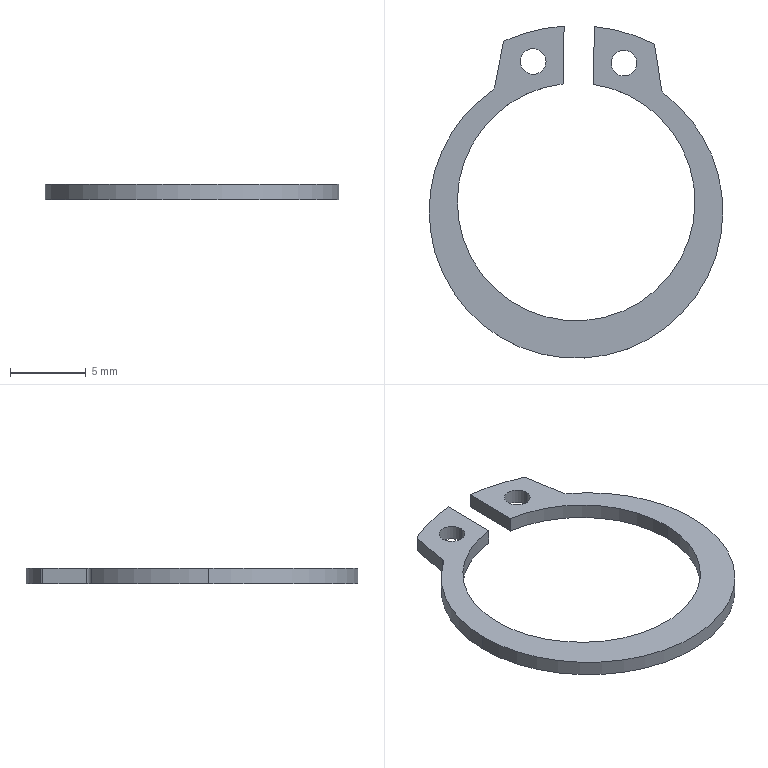Component | SolidWorks | HopperAssembly-1_20211103-210426-70669.STEP-1_-_-_-1.STEP-1_GB894_1-86_A_17.STEP-1 | 1 solid | 22 faces | box 19.4 x 21.94 x 1 mm | volume 118 mm3 | cylinder 16 | plane 6 | commonest cylinder face diameters 1.7 x4 19.4 x3 15.7 x3 1 x2 0.4 x2 23.3 x2
STEP:
#1=COLOUR_RGB('',0.7922,0.8196,0.9333);
#2=FILL_AREA_STYLE_COLOUR('',#1);
#3=FILL_AREA_STYLE('',(#2));
#4=SURFACE_STYLE_FILL_AREA(#3);
#5=SURFACE_SIDE_STYLE('',(#4));
#6=SURFACE_STYLE_USAGE(.BOTH.,#5);
#7=PRESENTATION_STYLE_ASSIGNMENT((#6));
#8=CARTESIAN_POINT('',(-104.551,33.416,-15.649));
#9=VERTEX_POINT('',#8);
#10=CARTESIAN_POINT('',(-104.484,33.414,-15.649));
#11=VERTEX_POINT('',#10);
#12=CARTESIAN_POINT('',(-104.517,33.415,-15.649));
#13=DIRECTION('',(0.,0.,-1.));
#14=DIRECTION('',(0.9998,-0.01747,0.));
#15=AXIS2_PLACEMENT_3D('',#12,#13,#14);
#16=CIRCLE('',#15,0.03346);
#17=EDGE_CURVE('',#9,#11,#16,.T.);
#18=ORIENTED_EDGE('',*,*,#17,.T.);
#19=CARTESIAN_POINT('',(-104.517,33.415,-15.649));
#20=DIRECTION('',(0.,0.,-1.));
#21=DIRECTION('',(0.9998,-0.01747,0.));
#22=AXIS2_PLACEMENT_3D('',#19,#20,#21);
#23=CIRCLE('',#22,0.03346);
#24=EDGE_CURVE('',#11,#9,#23,.T.);
#25=ORIENTED_EDGE('',*,*,#24,.T.);
#26=EDGE_LOOP('',(#18,#25));
#27=FACE_BOUND('',#26,.T.);
#28=CARTESIAN_POINT('',(-104.315,33.411,-15.649));
#29=VERTEX_POINT('',#28);
#30=CARTESIAN_POINT('',(-104.248,33.41,-15.649));
#31=VERTEX_POINT('',#30);
#32=CARTESIAN_POINT('',(-104.281,33.411,-15.649));
#33=DIRECTION('',(0.,0.,-1.));
#34=DIRECTION('',(-0.9998,0.01747,0.));
#35=AXIS2_PLACEMENT_3D('',#32,#33,#34);
#36=CIRCLE('',#35,0.03346);
#37=EDGE_CURVE('',#29,#31,#36,.T.);
#38=ORIENTED_EDGE('',*,*,#37,.T.);
#39=CARTESIAN_POINT('',(-104.281,33.411,-15.649));
#40=DIRECTION('',(0.,0.,-1.));
#41=DIRECTION('',(-0.9998,0.01747,0.));
#42=AXIS2_PLACEMENT_3D('',#39,#40,#41);
#43=CIRCLE('',#42,0.03346);
#44=EDGE_CURVE('',#31,#29,#43,.T.);
#45=ORIENTED_EDGE('',*,*,#44,.T.);
#46=EDGE_LOOP('',(#38,#45));
#47=FACE_BOUND('',#46,.T.);
#48=CARTESIAN_POINT('',(-104.625,33.338,-15.649));
#49=VERTEX_POINT('',#48);
#50=CARTESIAN_POINT('',(-104.617,33.35,-15.649));
#51=VERTEX_POINT('',#50);
#52=CARTESIAN_POINT('',(-104.637,33.354,-15.649));
#53=DIRECTION('',(-0.,-0.,1.));
#54=DIRECTION('',(0.9998,-0.01747,0.));
#55=AXIS2_PLACEMENT_3D('',#52,#53,#54);
#56=CIRCLE('',#55,0.01969);
#57=EDGE_CURVE('',#49,#51,#56,.T.);
#58=ORIENTED_EDGE('',*,*,#57,.F.);
#59=CARTESIAN_POINT('',(-104.788,33.032,-15.649));
#60=VERTEX_POINT('',#59);
#61=CARTESIAN_POINT('',(-104.406,33.025,-15.649));
#62=DIRECTION('',(0.,0.,-1.));
#63=DIRECTION('',(0.9998,-0.01747,0.));
#64=AXIS2_PLACEMENT_3D('',#61,#62,#63);
#65=CIRCLE('',#64,0.3819);
#66=EDGE_CURVE('',#60,#49,#65,.T.);
#67=ORIENTED_EDGE('',*,*,#66,.F.);
#68=CARTESIAN_POINT('',(-104.024,33.019,-15.649));
#69=VERTEX_POINT('',#68);
#70=CARTESIAN_POINT('',(-104.406,33.025,-15.649));
#71=DIRECTION('',(0.,0.,-1.));
#72=DIRECTION('',(0.9998,-0.01747,0.));
#73=AXIS2_PLACEMENT_3D('',#70,#71,#72);
#74=CIRCLE('',#73,0.3819);
#75=EDGE_CURVE('',#69,#60,#74,.T.);
#76=ORIENTED_EDGE('',*,*,#75,.F.);
#77=CARTESIAN_POINT('',(-104.176,33.33,-15.649));
#78=VERTEX_POINT('',#77);
#79=CARTESIAN_POINT('',(-104.406,33.025,-15.649));
#80=DIRECTION('',(0.,0.,-1.));
#81=DIRECTION('',(0.9998,-0.01747,0.));
#82=AXIS2_PLACEMENT_3D('',#79,#80,#81);
#83=CIRCLE('',#82,0.3819);
#84=EDGE_CURVE('',#78,#69,#83,.T.);
#85=ORIENTED_EDGE('',*,*,#84,.F.);
#86=CARTESIAN_POINT('',(-104.184,33.343,-15.649));
#87=VERTEX_POINT('',#86);
#88=CARTESIAN_POINT('',(-104.164,33.346,-15.649));
#89=DIRECTION('',(-0.,-0.,1.));
#90=DIRECTION('',(-0.9998,0.01747,0.));
#91=AXIS2_PLACEMENT_3D('',#88,#89,#90);
#92=CIRCLE('',#91,0.01969);
#93=EDGE_CURVE('',#87,#78,#92,.T.);
#94=ORIENTED_EDGE('',*,*,#93,.F.);
#95=CARTESIAN_POINT('',(-104.202,33.457,-15.649));
#96=VERTEX_POINT('',#95);
#97=CARTESIAN_POINT('',(-104.184,33.343,-15.649));
#98=DIRECTION('',(0.1564,-0.9877,-0.));
#99=VECTOR('',#98,39.37);
#100=LINE('',#97,#99);
#101=EDGE_CURVE('',#96,#87,#100,.T.);
#102=ORIENTED_EDGE('',*,*,#101,.F.);
#103=CARTESIAN_POINT('',(-104.206,33.463,-15.649));
#104=VERTEX_POINT('',#103);
#105=CARTESIAN_POINT('',(-104.209,33.456,-15.649));
#106=DIRECTION('',(0.,0.,-1.));
#107=DIRECTION('',(0.9998,-0.01747,0.));
#108=AXIS2_PLACEMENT_3D('',#105,#106,#107);
#109=CIRCLE('',#108,0.007874);
#110=EDGE_CURVE('',#104,#96,#109,.T.);
#111=ORIENTED_EDGE('',*,*,#110,.F.);
#112=CARTESIAN_POINT('',(-104.358,33.506,-15.649));
#113=VERTEX_POINT('',#112);
#114=CARTESIAN_POINT('',(-104.406,33.05,-15.649));
#115=DIRECTION('',(0.,0.,-1.));
#116=DIRECTION('',(0.9998,-0.01747,0.));
#117=AXIS2_PLACEMENT_3D('',#114,#115,#116);
#118=CIRCLE('',#117,0.4587);
#119=EDGE_CURVE('',#113,#104,#118,.T.);
#120=ORIENTED_EDGE('',*,*,#119,.F.);
#121=CARTESIAN_POINT('',(-104.361,33.356,-15.649));
#122=VERTEX_POINT('',#121);
#123=CARTESIAN_POINT('',(-104.361,33.356,-15.649));
#124=DIRECTION('',(0.01747,0.9998,0.));
#125=VECTOR('',#124,39.37);
#126=LINE('',#123,#125);
#127=EDGE_CURVE('',#122,#113,#126,.T.);
#128=ORIENTED_EDGE('',*,*,#127,.F.);
#129=CARTESIAN_POINT('',(-104.097,33.044,-15.649));
#130=VERTEX_POINT('',#129);
#131=CARTESIAN_POINT('',(-104.406,33.05,-15.649));
#132=DIRECTION('',(-0.,-0.,1.));
#133=DIRECTION('',(0.9998,-0.01747,0.));
#134=AXIS2_PLACEMENT_3D('',#131,#132,#133);
#135=CIRCLE('',#134,0.3091);
#136=EDGE_CURVE('',#130,#122,#135,.T.);
#137=ORIENTED_EDGE('',*,*,#136,.F.);
#138=CARTESIAN_POINT('',(-104.715,33.055,-15.649));
#139=VERTEX_POINT('',#138);
#140=CARTESIAN_POINT('',(-104.406,33.05,-15.649));
#141=DIRECTION('',(-0.,-0.,1.));
#142=DIRECTION('',(0.9998,-0.01747,0.));
#143=AXIS2_PLACEMENT_3D('',#140,#141,#142);
#144=CIRCLE('',#143,0.3091);
#145=EDGE_CURVE('',#139,#130,#144,.T.);
#146=ORIENTED_EDGE('',*,*,#145,.F.);
#147=CARTESIAN_POINT('',(-104.44,33.357,-15.649));
#148=VERTEX_POINT('',#147);
#149=CARTESIAN_POINT('',(-104.406,33.05,-15.649));
#150=DIRECTION('',(-0.,-0.,1.));
#151=DIRECTION('',(0.9998,-0.01747,0.));
#152=AXIS2_PLACEMENT_3D('',#149,#150,#151);
#153=CIRCLE('',#152,0.3091);
#154=EDGE_CURVE('',#148,#139,#153,.T.);
#155=ORIENTED_EDGE('',*,*,#154,.F.);
#156=CARTESIAN_POINT('',(-104.437,33.507,-15.649));
#157=VERTEX_POINT('',#156);
#158=CARTESIAN_POINT('',(-104.44,33.357,-15.649));
#159=DIRECTION('',(-0.01747,-0.9998,-0.));
#160=VECTOR('',#159,39.37);
#161=LINE('',#158,#160);
#162=EDGE_CURVE('',#157,#148,#161,.T.);
#163=ORIENTED_EDGE('',*,*,#162,.F.);
#164=CARTESIAN_POINT('',(-104.591,33.469,-15.649));
#165=VERTEX_POINT('',#164);
#166=CARTESIAN_POINT('',(-104.406,33.05,-15.649));
#167=DIRECTION('',(0.,0.,-1.));
#168=DIRECTION('',(-0.9998,0.01747,0.));
#169=AXIS2_PLACEMENT_3D('',#166,#167,#168);
#170=CIRCLE('',#169,0.4587);
#171=EDGE_CURVE('',#165,#157,#170,.T.);
#172=ORIENTED_EDGE('',*,*,#171,.F.);
#173=CARTESIAN_POINT('',(-104.595,33.464,-15.649));
#174=VERTEX_POINT('',#173);
#175=CARTESIAN_POINT('',(-104.588,33.462,-15.649));
#176=DIRECTION('',(0.,0.,-1.));
#177=DIRECTION('',(-0.9998,0.01747,0.));
#178=AXIS2_PLACEMENT_3D('',#175,#176,#177);
#179=CIRCLE('',#178,0.007874);
#180=EDGE_CURVE('',#174,#165,#179,.T.);
#181=ORIENTED_EDGE('',*,*,#180,.F.);
#182=CARTESIAN_POINT('',(-104.617,33.35,-15.649));
#183=DIRECTION('',(0.1908,0.9816,0.));
#184=VECTOR('',#183,39.37);
#185=LINE('',#182,#184);
#186=EDGE_CURVE('',#51,#174,#185,.T.);
#187=ORIENTED_EDGE('',*,*,#186,.F.);
#188=EDGE_LOOP('',(#58,#67,#76,#85,#94,#102,#111,#120,#128,#137,#146,#155,#163,#172,#181,#187));
#189=FACE_OUTER_BOUND('',#188,.T.);
#190=CARTESIAN_POINT('',(-104.637,33.354,-15.649));
#191=DIRECTION('',(0.,0.,-1.));
#192=DIRECTION('',(0.9998,-0.01747,0.));
#193=AXIS2_PLACEMENT_3D('',#190,#191,#192);
#194=PLANE('',#193);
#195=ADVANCED_FACE('',(#27,#47,#189),#194,.F.);
#196=CARTESIAN_POINT('',(-104.248,33.41,-15.688));
#197=VERTEX_POINT('',#196);
#198=CARTESIAN_POINT('',(-104.248,33.41,-15.688));
#199=DIRECTION('',(-0.,-0.,1.));
#200=VECTOR('',#199,39.37);
#201=LINE('',#198,#200);
#202=EDGE_CURVE('',#197,#31,#201,.T.);
#203=ORIENTED_EDGE('',*,*,#202,.F.);
#204=CARTESIAN_POINT('',(-104.315,33.411,-15.688));
#205=VERTEX_POINT('',#204);
#206=CARTESIAN_POINT('',(-104.281,33.411,-15.688));
#207=DIRECTION('',(0.,0.,-1.));
#208=DIRECTION('',(-0.9998,0.01747,0.));
#209=AXIS2_PLACEMENT_3D('',#206,#207,#208);
#210=CIRCLE('',#209,0.03346);
#211=EDGE_CURVE('',#197,#205,#210,.T.);
#212=ORIENTED_EDGE('',*,*,#211,.T.);
#213=CARTESIAN_POINT('',(-104.315,33.411,-15.688));
#214=DIRECTION('',(-0.,-0.,1.));
#215=VECTOR('',#214,39.37);
#216=LINE('',#213,#215);
#217=EDGE_CURVE('',#205,#29,#216,.T.);
#218=ORIENTED_EDGE('',*,*,#217,.T.);
#219=ORIENTED_EDGE('',*,*,#44,.F.);
#220=EDGE_LOOP('',(#203,#212,#218,#219));
#221=FACE_OUTER_BOUND('',#220,.T.);
#222=CARTESIAN_POINT('',(-104.281,33.411,-15.688));
#223=DIRECTION('',(-0.,-0.,1.));
#224=DIRECTION('',(-0.9998,0.01747,0.));
#225=AXIS2_PLACEMENT_3D('',#222,#223,#224);
#226=CYLINDRICAL_SURFACE('',#225,0.03346);
#227=ADVANCED_FACE('',(#221),#226,.F.);
#228=CARTESIAN_POINT('',(-104.484,33.414,-15.688));
#229=VERTEX_POINT('',#228);
#230=CARTESIAN_POINT('',(-104.484,33.414,-15.688));
#231=DIRECTION('',(-0.,-0.,1.));
#232=VECTOR('',#231,39.37);
#233=LINE('',#230,#232);
#234=EDGE_CURVE('',#229,#11,#233,.T.);
#235=ORIENTED_EDGE('',*,*,#234,.F.);
#236=CARTESIAN_POINT('',(-104.551,33.416,-15.688));
#237=VERTEX_POINT('',#236);
#238=CARTESIAN_POINT('',(-104.517,33.415,-15.688));
#239=DIRECTION('',(0.,0.,-1.));
#240=DIRECTION('',(0.9998,-0.01747,0.));
#241=AXIS2_PLACEMENT_3D('',#238,#239,#240);
#242=CIRCLE('',#241,0.03346);
#243=EDGE_CURVE('',#229,#237,#242,.T.);
#244=ORIENTED_EDGE('',*,*,#243,.T.);
#245=CARTESIAN_POINT('',(-104.551,33.416,-15.688));
#246=DIRECTION('',(-0.,-0.,1.));
#247=VECTOR('',#246,39.37);
#248=LINE('',#245,#247);
#249=EDGE_CURVE('',#237,#9,#248,.T.);
#250=ORIENTED_EDGE('',*,*,#249,.T.);
#251=ORIENTED_EDGE('',*,*,#24,.F.);
#252=EDGE_LOOP('',(#235,#244,#250,#251));
#253=FACE_OUTER_BOUND('',#252,.T.);
#254=CARTESIAN_POINT('',(-104.517,33.415,-15.688));
#255=DIRECTION('',(-0.,-0.,1.));
#256=DIRECTION('',(-0.9998,0.01747,0.));
#257=AXIS2_PLACEMENT_3D('',#254,#255,#256);
#258=CYLINDRICAL_SURFACE('',#257,0.03346);
#259=ADVANCED_FACE('',(#253),#258,.F.);
#260=CARTESIAN_POINT('',(-104.024,33.019,-15.688));
#261=VERTEX_POINT('',#260);
#262=CARTESIAN_POINT('',(-104.024,33.019,-15.688));
#263=DIRECTION('',(-0.,-0.,1.));
#264=VECTOR('',#263,39.37);
#265=LINE('',#262,#264);
#266=EDGE_CURVE('',#261,#69,#265,.T.);
#267=ORIENTED_EDGE('',*,*,#266,.F.);
#268=CARTESIAN_POINT('',(-104.176,33.33,-15.688));
#269=VERTEX_POINT('',#268);
#270=CARTESIAN_POINT('',(-104.406,33.025,-15.688));
#271=DIRECTION('',(0.,0.,-1.));
#272=DIRECTION('',(0.9998,-0.01747,0.));
#273=AXIS2_PLACEMENT_3D('',#270,#271,#272);
#274=CIRCLE('',#273,0.3819);
#275=EDGE_CURVE('',#269,#261,#274,.T.);
#276=ORIENTED_EDGE('',*,*,#275,.F.);
#277=CARTESIAN_POINT('',(-104.176,33.33,-15.688));
#278=DIRECTION('',(-0.,-0.,1.));
#279=VECTOR('',#278,39.37);
#280=LINE('',#277,#279);
#281=EDGE_CURVE('',#269,#78,#280,.T.);
#282=ORIENTED_EDGE('',*,*,#281,.T.);
#283=ORIENTED_EDGE('',*,*,#84,.T.);
#284=EDGE_LOOP('',(#267,#276,#282,#283));
#285=FACE_OUTER_BOUND('',#284,.T.);
#286=CARTESIAN_POINT('',(-104.406,33.025,-15.688));
#287=DIRECTION('',(-0.,-0.,1.));
#288=DIRECTION('',(-0.9998,0.01747,0.));
#289=AXIS2_PLACEMENT_3D('',#286,#287,#288);
#290=CYLINDRICAL_SURFACE('',#289,0.3819);
#291=ADVANCED_FACE('',(#285),#290,.T.);
#292=CARTESIAN_POINT('',(-104.184,33.343,-15.688));
#293=VERTEX_POINT('',#292);
#294=CARTESIAN_POINT('',(-104.184,33.343,-15.688));
#295=DIRECTION('',(-0.,-0.,1.));
#296=VECTOR('',#295,39.37);
#297=LINE('',#294,#296);
#298=EDGE_CURVE('',#293,#87,#297,.T.);
#299=ORIENTED_EDGE('',*,*,#298,.T.);
#300=ORIENTED_EDGE('',*,*,#93,.T.);
#301=ORIENTED_EDGE('',*,*,#281,.F.);
#302=CARTESIAN_POINT('',(-104.164,33.346,-15.688));
#303=DIRECTION('',(-0.,-0.,1.));
#304=DIRECTION('',(-0.9998,0.01747,0.));
#305=AXIS2_PLACEMENT_3D('',#302,#303,#304);
#306=CIRCLE('',#305,0.01969);
#307=EDGE_CURVE('',#293,#269,#306,.T.);
#308=ORIENTED_EDGE('',*,*,#307,.F.);
#309=EDGE_LOOP('',(#299,#300,#301,#308));
#310=FACE_OUTER_BOUND('',#309,.T.);
#311=CARTESIAN_POINT('',(-104.164,33.346,-15.688));
#312=DIRECTION('',(-0.,-0.,1.));
#313=DIRECTION('',(-0.9998,0.01747,0.));
#314=AXIS2_PLACEMENT_3D('',#311,#312,#313);
#315=CYLINDRICAL_SURFACE('',#314,0.01969);
#316=ADVANCED_FACE('',(#310),#315,.F.);
#317=CARTESIAN_POINT('',(-104.202,33.457,-15.688));
#318=VERTEX_POINT('',#317);
#319=CARTESIAN_POINT('',(-104.202,33.457,-15.688));
#320=DIRECTION('',(-0.,-0.,1.));
#321=VECTOR('',#320,39.37);
#322=LINE('',#319,#321);
#323=EDGE_CURVE('',#318,#96,#322,.T.);
#324=ORIENTED_EDGE('',*,*,#323,.T.);
#325=ORIENTED_EDGE('',*,*,#101,.T.);
#326=ORIENTED_EDGE('',*,*,#298,.F.);
#327=CARTESIAN_POINT('',(-104.184,33.343,-15.688));
#328=DIRECTION('',(0.1564,-0.9877,-0.));
#329=VECTOR('',#328,39.37);
#330=LINE('',#327,#329);
#331=EDGE_CURVE('',#318,#293,#330,.T.);
#332=ORIENTED_EDGE('',*,*,#331,.F.);
#333=EDGE_LOOP('',(#324,#325,#326,#332));
#334=FACE_OUTER_BOUND('',#333,.T.);
#335=CARTESIAN_POINT('',(-104.184,33.343,-15.688));
#336=DIRECTION('',(-0.9877,-0.1564,-0.));
#337=DIRECTION('',(0.,0.,-1.));
#338=AXIS2_PLACEMENT_3D('',#335,#336,#337);
#339=PLANE('',#338);
#340=ADVANCED_FACE('',(#334),#339,.F.);
#341=CARTESIAN_POINT('',(-104.206,33.463,-15.688));
#342=VERTEX_POINT('',#341);
#343=CARTESIAN_POINT('',(-104.206,33.463,-15.688));
#344=DIRECTION('',(-0.,-0.,1.));
#345=VECTOR('',#344,39.37);
#346=LINE('',#343,#345);
#347=EDGE_CURVE('',#342,#104,#346,.T.);
#348=ORIENTED_EDGE('',*,*,#347,.T.);
#349=ORIENTED_EDGE('',*,*,#110,.T.);
#350=ORIENTED_EDGE('',*,*,#323,.F.);
#351=CARTESIAN_POINT('',(-104.209,33.456,-15.688));
#352=DIRECTION('',(0.,0.,-1.));
#353=DIRECTION('',(0.9998,-0.01747,0.));
#354=AXIS2_PLACEMENT_3D('',#351,#352,#353);
#355=CIRCLE('',#354,0.007874);
#356=EDGE_CURVE('',#342,#318,#355,.T.);
#357=ORIENTED_EDGE('',*,*,#356,.F.);
#358=EDGE_LOOP('',(#348,#349,#350,#357));
#359=FACE_OUTER_BOUND('',#358,.T.);
#360=CARTESIAN_POINT('',(-104.209,33.456,-15.688));
#361=DIRECTION('',(-0.,-0.,1.));
#362=DIRECTION('',(-0.9998,0.01747,0.));
#363=AXIS2_PLACEMENT_3D('',#360,#361,#362);
#364=CYLINDRICAL_SURFACE('',#363,0.007874);
#365=ADVANCED_FACE('',(#359),#364,.T.);
#366=CARTESIAN_POINT('',(-104.358,33.506,-15.688));
#367=VERTEX_POINT('',#366);
#368=CARTESIAN_POINT('',(-104.358,33.506,-15.688));
#369=DIRECTION('',(-0.,-0.,1.));
#370=VECTOR('',#369,39.37);
#371=LINE('',#368,#370);
#372=EDGE_CURVE('',#367,#113,#371,.T.);
#373=ORIENTED_EDGE('',*,*,#372,.T.);
#374=ORIENTED_EDGE('',*,*,#119,.T.);
#375=ORIENTED_EDGE('',*,*,#347,.F.);
#376=CARTESIAN_POINT('',(-104.406,33.05,-15.688));
#377=DIRECTION('',(0.,0.,-1.));
#378=DIRECTION('',(0.9998,-0.01747,0.));
#379=AXIS2_PLACEMENT_3D('',#376,#377,#378);
#380=CIRCLE('',#379,0.4587);
#381=EDGE_CURVE('',#367,#342,#380,.T.);
#382=ORIENTED_EDGE('',*,*,#381,.F.);
#383=EDGE_LOOP('',(#373,#374,#375,#382));
#384=FACE_OUTER_BOUND('',#383,.T.);
#385=CARTESIAN_POINT('',(-104.406,33.05,-15.688));
#386=DIRECTION('',(-0.,-0.,1.));
#387=DIRECTION('',(-0.9998,0.01747,0.));
#388=AXIS2_PLACEMENT_3D('',#385,#386,#387);
#389=CYLINDRICAL_SURFACE('',#388,0.4587);
#390=ADVANCED_FACE('',(#384),#389,.T.);
#391=CARTESIAN_POINT('',(-104.361,33.356,-15.688));
#392=VERTEX_POINT('',#391);
#393=CARTESIAN_POINT('',(-104.361,33.356,-15.688));
#394=DIRECTION('',(-0.,-0.,1.));
#395=VECTOR('',#394,39.37);
#396=LINE('',#393,#395);
#397=EDGE_CURVE('',#392,#122,#396,.T.);
#398=ORIENTED_EDGE('',*,*,#397,.T.);
#399=ORIENTED_EDGE('',*,*,#127,.T.);
#400=ORIENTED_EDGE('',*,*,#372,.F.);
#401=CARTESIAN_POINT('',(-104.361,33.356,-15.688));
#402=DIRECTION('',(0.01747,0.9998,0.));
#403=VECTOR('',#402,39.37);
#404=LINE('',#401,#403);
#405=EDGE_CURVE('',#392,#367,#404,.T.);
#406=ORIENTED_EDGE('',*,*,#405,.F.);
#407=EDGE_LOOP('',(#398,#399,#400,#406));
#408=FACE_OUTER_BOUND('',#407,.T.);
#409=CARTESIAN_POINT('',(-104.361,33.356,-15.688));
#410=DIRECTION('',(0.9998,-0.01747,0.));
#411=DIRECTION('',(-0.01747,-0.9998,-0.));
#412=AXIS2_PLACEMENT_3D('',#409,#410,#411);
#413=PLANE('',#412);
#414=ADVANCED_FACE('',(#408),#413,.F.);
#415=CARTESIAN_POINT('',(-104.715,33.055,-15.688));
#416=VERTEX_POINT('',#415);
#417=CARTESIAN_POINT('',(-104.715,33.055,-15.688));
#418=DIRECTION('',(-0.,-0.,1.));
#419=VECTOR('',#418,39.37);
#420=LINE('',#417,#419);
#421=EDGE_CURVE('',#416,#139,#420,.T.);
#422=ORIENTED_EDGE('',*,*,#421,.F.);
#423=CARTESIAN_POINT('',(-104.44,33.357,-15.688));
#424=VERTEX_POINT('',#423);
#425=CARTESIAN_POINT('',(-104.406,33.05,-15.688));
#426=DIRECTION('',(-0.,-0.,1.));
#427=DIRECTION('',(0.9998,-0.01747,0.));
#428=AXIS2_PLACEMENT_3D('',#425,#426,#427);
#429=CIRCLE('',#428,0.3091);
#430=EDGE_CURVE('',#424,#416,#429,.T.);
#431=ORIENTED_EDGE('',*,*,#430,.F.);
#432=CARTESIAN_POINT('',(-104.44,33.357,-15.688));
#433=DIRECTION('',(-0.,-0.,1.));
#434=VECTOR('',#433,39.37);
#435=LINE('',#432,#434);
#436=EDGE_CURVE('',#424,#148,#435,.T.);
#437=ORIENTED_EDGE('',*,*,#436,.T.);
#438=ORIENTED_EDGE('',*,*,#154,.T.);
#439=EDGE_LOOP('',(#422,#431,#437,#438));
#440=FACE_OUTER_BOUND('',#439,.T.);
#441=CARTESIAN_POINT('',(-104.406,33.05,-15.688));
#442=DIRECTION('',(-0.,-0.,1.));
#443=DIRECTION('',(-0.9998,0.01747,0.));
#444=AXIS2_PLACEMENT_3D('',#441,#442,#443);
#445=CYLINDRICAL_SURFACE('',#444,0.3091);
#446=ADVANCED_FACE('',(#440),#445,.F.);
#447=CARTESIAN_POINT('',(-104.437,33.507,-15.688));
#448=VERTEX_POINT('',#447);
#449=CARTESIAN_POINT('',(-104.437,33.507,-15.688));
#450=DIRECTION('',(-0.,-0.,1.));
#451=VECTOR('',#450,39.37);
#452=LINE('',#449,#451);
#453=EDGE_CURVE('',#448,#157,#452,.T.);
#454=ORIENTED_EDGE('',*,*,#453,.T.);
#455=ORIENTED_EDGE('',*,*,#162,.T.);
#456=ORIENTED_EDGE('',*,*,#436,.F.);
#457=CARTESIAN_POINT('',(-104.44,33.357,-15.688));
#458=DIRECTION('',(-0.01747,-0.9998,-0.));
#459=VECTOR('',#458,39.37);
#460=LINE('',#457,#459);
#461=EDGE_CURVE('',#448,#424,#460,.T.);
#462=ORIENTED_EDGE('',*,*,#461,.F.);
#463=EDGE_LOOP('',(#454,#455,#456,#462));
#464=FACE_OUTER_BOUND('',#463,.T.);
#465=CARTESIAN_POINT('',(-104.44,33.357,-15.688));
#466=DIRECTION('',(-0.9998,0.01747,-0.));
#467=DIRECTION('',(-0.01747,-0.9998,-0.));
#468=AXIS2_PLACEMENT_3D('',#465,#466,#467);
#469=PLANE('',#468);
#470=ADVANCED_FACE('',(#464),#469,.F.);
#471=CARTESIAN_POINT('',(-104.591,33.469,-15.688));
#472=VERTEX_POINT('',#471);
#473=CARTESIAN_POINT('',(-104.591,33.469,-15.688));
#474=DIRECTION('',(-0.,-0.,1.));
#475=VECTOR('',#474,39.37);
#476=LINE('',#473,#475);
#477=EDGE_CURVE('',#472,#165,#476,.T.);
#478=ORIENTED_EDGE('',*,*,#477,.T.);
#479=ORIENTED_EDGE('',*,*,#171,.T.);
#480=ORIENTED_EDGE('',*,*,#453,.F.);
#481=CARTESIAN_POINT('',(-104.406,33.05,-15.688));
#482=DIRECTION('',(0.,0.,-1.));
#483=DIRECTION('',(-0.9998,0.01747,0.));
#484=AXIS2_PLACEMENT_3D('',#481,#482,#483);
#485=CIRCLE('',#484,0.4587);
#486=EDGE_CURVE('',#472,#448,#485,.T.);
#487=ORIENTED_EDGE('',*,*,#486,.F.);
#488=EDGE_LOOP('',(#478,#479,#480,#487));
#489=FACE_OUTER_BOUND('',#488,.T.);
#490=CARTESIAN_POINT('',(-104.406,33.05,-15.688));
#491=DIRECTION('',(-0.,-0.,1.));
#492=DIRECTION('',(-0.9998,0.01747,0.));
#493=AXIS2_PLACEMENT_3D('',#490,#491,#492);
#494=CYLINDRICAL_SURFACE('',#493,0.4587);
#495=ADVANCED_FACE('',(#489),#494,.T.);
#496=CARTESIAN_POINT('',(-104.595,33.464,-15.688));
#497=VERTEX_POINT('',#496);
#498=CARTESIAN_POINT('',(-104.595,33.464,-15.688));
#499=DIRECTION('',(-0.,-0.,1.));
#500=VECTOR('',#499,39.37);
#501=LINE('',#498,#500);
#502=EDGE_CURVE('',#497,#174,#501,.T.);
#503=ORIENTED_EDGE('',*,*,#502,.T.);
#504=ORIENTED_EDGE('',*,*,#180,.T.);
#505=ORIENTED_EDGE('',*,*,#477,.F.);
#506=CARTESIAN_POINT('',(-104.588,33.462,-15.688));
#507=DIRECTION('',(0.,0.,-1.));
#508=DIRECTION('',(-0.9998,0.01747,0.));
#509=AXIS2_PLACEMENT_3D('',#506,#507,#508);
#510=CIRCLE('',#509,0.007874);
#511=EDGE_CURVE('',#497,#472,#510,.T.);
#512=ORIENTED_EDGE('',*,*,#511,.F.);
#513=EDGE_LOOP('',(#503,#504,#505,#512));
#514=FACE_OUTER_BOUND('',#513,.T.);
#515=CARTESIAN_POINT('',(-104.588,33.462,-15.688));
#516=DIRECTION('',(-0.,-0.,1.));
#517=DIRECTION('',(-0.9998,0.01747,0.));
#518=AXIS2_PLACEMENT_3D('',#515,#516,#517);
#519=CYLINDRICAL_SURFACE('',#518,0.007874);
#520=ADVANCED_FACE('',(#514),#519,.T.);
#521=CARTESIAN_POINT('',(-104.617,33.35,-15.688));
#522=VERTEX_POINT('',#521);
#523=CARTESIAN_POINT('',(-104.617,33.35,-15.688));
#524=DIRECTION('',(-0.,-0.,1.));
#525=VECTOR('',#524,39.37);
#526=LINE('',#523,#525);
#527=EDGE_CURVE('',#522,#51,#526,.T.);
#528=ORIENTED_EDGE('',*,*,#527,.T.);
#529=ORIENTED_EDGE('',*,*,#186,.T.);
#530=ORIENTED_EDGE('',*,*,#502,.F.);
#531=CARTESIAN_POINT('',(-104.617,33.35,-15.688));
#532=DIRECTION('',(0.1908,0.9816,0.));
#533=VECTOR('',#532,39.37);
#534=LINE('',#531,#533);
#535=EDGE_CURVE('',#522,#497,#534,.T.);
#536=ORIENTED_EDGE('',*,*,#535,.F.);
#537=EDGE_LOOP('',(#528,#529,#530,#536));
#538=FACE_OUTER_BOUND('',#537,.T.);
#539=CARTESIAN_POINT('',(-104.617,33.35,-15.688));
#540=DIRECTION('',(0.9816,-0.1908,0.));
#541=DIRECTION('',(-0.,-0.,1.));
#542=AXIS2_PLACEMENT_3D('',#539,#540,#541);
#543=PLANE('',#542);
#544=ADVANCED_FACE('',(#538),#543,.F.);
#545=CARTESIAN_POINT('',(-104.625,33.338,-15.688));
#546=VERTEX_POINT('',#545);
#547=CARTESIAN_POINT('',(-104.625,33.338,-15.688));
#548=DIRECTION('',(-0.,-0.,1.));
#549=VECTOR('',#548,39.37);
#550=LINE('',#547,#549);
#551=EDGE_CURVE('',#546,#49,#550,.T.);
#552=ORIENTED_EDGE('',*,*,#551,.T.);
#553=ORIENTED_EDGE('',*,*,#57,.T.);
#554=ORIENTED_EDGE('',*,*,#527,.F.);
#555=CARTESIAN_POINT('',(-104.637,33.354,-15.688));
#556=DIRECTION('',(-0.,-0.,1.));
#557=DIRECTION('',(0.9998,-0.01747,0.));
#558=AXIS2_PLACEMENT_3D('',#555,#556,#557);
#559=CIRCLE('',#558,0.01969);
#560=EDGE_CURVE('',#546,#522,#559,.T.);
#561=ORIENTED_EDGE('',*,*,#560,.F.);
#562=EDGE_LOOP('',(#552,#553,#554,#561));
#563=FACE_OUTER_BOUND('',#562,.T.);
#564=CARTESIAN_POINT('',(-104.637,33.354,-15.688));
#565=DIRECTION('',(-0.,-0.,1.));
#566=DIRECTION('',(-0.9998,0.01747,0.));
#567=AXIS2_PLACEMENT_3D('',#564,#565,#566);
#568=CYLINDRICAL_SURFACE('',#567,0.01969);
#569=ADVANCED_FACE('',(#563),#568,.F.);
#570=CARTESIAN_POINT('',(-104.281,33.411,-15.688));
#571=DIRECTION('',(0.,0.,-1.));
#572=DIRECTION('',(-0.9998,0.01747,0.));
#573=AXIS2_PLACEMENT_3D('',#570,#571,#572);
#574=CIRCLE('',#573,0.03346);
#575=EDGE_CURVE('',#205,#197,#574,.T.);
#576=ORIENTED_EDGE('',*,*,#575,.F.);
#577=ORIENTED_EDGE('',*,*,#211,.F.);
#578=EDGE_LOOP('',(#576,#577));
#579=FACE_BOUND('',#578,.T.);
#580=CARTESIAN_POINT('',(-104.517,33.415,-15.688));
#581=DIRECTION('',(0.,0.,-1.));
#582=DIRECTION('',(0.9998,-0.01747,0.));
#583=AXIS2_PLACEMENT_3D('',#580,#581,#582);
#584=CIRCLE('',#583,0.03346);
#585=EDGE_CURVE('',#237,#229,#584,.T.);
#586=ORIENTED_EDGE('',*,*,#585,.F.);
#587=ORIENTED_EDGE('',*,*,#243,.F.);
#588=EDGE_LOOP('',(#586,#587));
#589=FACE_BOUND('',#588,.T.);
#590=ORIENTED_EDGE('',*,*,#560,.T.);
#591=ORIENTED_EDGE('',*,*,#535,.T.);
#592=ORIENTED_EDGE('',*,*,#511,.T.);
#593=ORIENTED_EDGE('',*,*,#486,.T.);
#594=ORIENTED_EDGE('',*,*,#461,.T.);
#595=ORIENTED_EDGE('',*,*,#430,.T.);
#596=CARTESIAN_POINT('',(-104.097,33.044,-15.688));
#597=VERTEX_POINT('',#596);
#598=CARTESIAN_POINT('',(-104.406,33.05,-15.688));
#599=DIRECTION('',(-0.,-0.,1.));
#600=DIRECTION('',(0.9998,-0.01747,0.));
#601=AXIS2_PLACEMENT_3D('',#598,#599,#600);
#602=CIRCLE('',#601,0.3091);
#603=EDGE_CURVE('',#416,#597,#602,.T.);
#604=ORIENTED_EDGE('',*,*,#603,.T.);
#605=CARTESIAN_POINT('',(-104.406,33.05,-15.688));
#606=DIRECTION('',(-0.,-0.,1.));
#607=DIRECTION('',(0.9998,-0.01747,0.));
#608=AXIS2_PLACEMENT_3D('',#605,#606,#607);
#609=CIRCLE('',#608,0.3091);
#610=EDGE_CURVE('',#597,#392,#609,.T.);
#611=ORIENTED_EDGE('',*,*,#610,.T.);
#612=ORIENTED_EDGE('',*,*,#405,.T.);
#613=ORIENTED_EDGE('',*,*,#381,.T.);
#614=ORIENTED_EDGE('',*,*,#356,.T.);
#615=ORIENTED_EDGE('',*,*,#331,.T.);
#616=ORIENTED_EDGE('',*,*,#307,.T.);
#617=ORIENTED_EDGE('',*,*,#275,.T.);
#618=CARTESIAN_POINT('',(-104.788,33.032,-15.688));
#619=VERTEX_POINT('',#618);
#620=CARTESIAN_POINT('',(-104.406,33.025,-15.688));
#621=DIRECTION('',(0.,0.,-1.));
#622=DIRECTION('',(0.9998,-0.01747,0.));
#623=AXIS2_PLACEMENT_3D('',#620,#621,#622);
#624=CIRCLE('',#623,0.3819);
#625=EDGE_CURVE('',#261,#619,#624,.T.);
#626=ORIENTED_EDGE('',*,*,#625,.T.);
#627=CARTESIAN_POINT('',(-104.406,33.025,-15.688));
#628=DIRECTION('',(0.,0.,-1.));
#629=DIRECTION('',(0.9998,-0.01747,0.));
#630=AXIS2_PLACEMENT_3D('',#627,#628,#629);
#631=CIRCLE('',#630,0.3819);
#632=EDGE_CURVE('',#619,#546,#631,.T.);
#633=ORIENTED_EDGE('',*,*,#632,.T.);
#634=EDGE_LOOP('',(#590,#591,#592,#593,#594,#595,#604,#611,#612,#613,#614,#615,#616,#617,#626,#633));
#635=FACE_OUTER_BOUND('',#634,.T.);
#636=CARTESIAN_POINT('',(-104.637,33.354,-15.688));
#637=DIRECTION('',(0.,0.,-1.));
#638=DIRECTION('',(0.9998,-0.01747,0.));
#639=AXIS2_PLACEMENT_3D('',#636,#637,#638);
#640=PLANE('',#639);
#641=ADVANCED_FACE('',(#579,#589,#635),#640,.T.);
#642=CARTESIAN_POINT('',(-104.097,33.044,-15.688));
#643=DIRECTION('',(-0.,-0.,1.));
#644=VECTOR('',#643,39.37);
#645=LINE('',#642,#644);
#646=EDGE_CURVE('',#597,#130,#645,.T.);
#647=ORIENTED_EDGE('',*,*,#646,.F.);
#648=ORIENTED_EDGE('',*,*,#603,.F.);
#649=ORIENTED_EDGE('',*,*,#421,.T.);
#650=ORIENTED_EDGE('',*,*,#145,.T.);
#651=EDGE_LOOP('',(#647,#648,#649,#650));
#652=FACE_OUTER_BOUND('',#651,.T.);
#653=CARTESIAN_POINT('',(-104.406,33.05,-15.688));
#654=DIRECTION('',(-0.,-0.,1.));
#655=DIRECTION('',(-0.9998,0.01747,0.));
#656=AXIS2_PLACEMENT_3D('',#653,#654,#655);
#657=CYLINDRICAL_SURFACE('',#656,0.3091);
#658=ADVANCED_FACE('',(#652),#657,.F.);
#659=ORIENTED_EDGE('',*,*,#610,.F.);
#660=ORIENTED_EDGE('',*,*,#646,.T.);
#661=ORIENTED_EDGE('',*,*,#136,.T.);
#662=ORIENTED_EDGE('',*,*,#397,.F.);
#663=EDGE_LOOP('',(#659,#660,#661,#662));
#664=FACE_OUTER_BOUND('',#663,.T.);
#665=CARTESIAN_POINT('',(-104.406,33.05,-15.688));
#666=DIRECTION('',(-0.,-0.,1.));
#667=DIRECTION('',(-0.9998,0.01747,0.));
#668=AXIS2_PLACEMENT_3D('',#665,#666,#667);
#669=CYLINDRICAL_SURFACE('',#668,0.3091);
#670=ADVANCED_FACE('',(#664),#669,.F.);
#671=ORIENTED_EDGE('',*,*,#632,.F.);
#672=CARTESIAN_POINT('',(-104.788,33.032,-15.688));
#673=DIRECTION('',(-0.,-0.,1.));
#674=VECTOR('',#673,39.37);
#675=LINE('',#672,#674);
#676=EDGE_CURVE('',#619,#60,#675,.T.);
#677=ORIENTED_EDGE('',*,*,#676,.T.);
#678=ORIENTED_EDGE('',*,*,#66,.T.);
#679=ORIENTED_EDGE('',*,*,#551,.F.);
#680=EDGE_LOOP('',(#671,#677,#678,#679));
#681=FACE_OUTER_BOUND('',#680,.T.);
#682=CARTESIAN_POINT('',(-104.406,33.025,-15.688));
#683=DIRECTION('',(-0.,-0.,1.));
#684=DIRECTION('',(-0.9998,0.01747,0.));
#685=AXIS2_PLACEMENT_3D('',#682,#683,#684);
#686=CYLINDRICAL_SURFACE('',#685,0.3819);
#687=ADVANCED_FACE('',(#681),#686,.T.);
#688=ORIENTED_EDGE('',*,*,#625,.F.);
#689=ORIENTED_EDGE('',*,*,#266,.T.);
#690=ORIENTED_EDGE('',*,*,#75,.T.);
#691=ORIENTED_EDGE('',*,*,#676,.F.);
#692=EDGE_LOOP('',(#688,#689,#690,#691));
#693=FACE_OUTER_BOUND('',#692,.T.);
#694=CARTESIAN_POINT('',(-104.406,33.025,-15.688));
#695=DIRECTION('',(-0.,-0.,1.));
#696=DIRECTION('',(-0.9998,0.01747,0.));
#697=AXIS2_PLACEMENT_3D('',#694,#695,#696);
#698=CYLINDRICAL_SURFACE('',#697,0.3819);
#699=ADVANCED_FACE('',(#693),#698,.T.);
#700=ORIENTED_EDGE('',*,*,#585,.T.);
#701=ORIENTED_EDGE('',*,*,#234,.T.);
#702=ORIENTED_EDGE('',*,*,#17,.F.);
#703=ORIENTED_EDGE('',*,*,#249,.F.);
#704=EDGE_LOOP('',(#700,#701,#702,#703));
#705=FACE_OUTER_BOUND('',#704,.T.);
#706=CARTESIAN_POINT('',(-104.517,33.415,-15.688));
#707=DIRECTION('',(-0.,-0.,1.));
#708=DIRECTION('',(-0.9998,0.01747,0.));
#709=AXIS2_PLACEMENT_3D('',#706,#707,#708);
#710=CYLINDRICAL_SURFACE('',#709,0.03346);
#711=ADVANCED_FACE('',(#705),#710,.F.);
#712=ORIENTED_EDGE('',*,*,#575,.T.);
#713=ORIENTED_EDGE('',*,*,#202,.T.);
#714=ORIENTED_EDGE('',*,*,#37,.F.);
#715=ORIENTED_EDGE('',*,*,#217,.F.);
#716=EDGE_LOOP('',(#712,#713,#714,#715));
#717=FACE_OUTER_BOUND('',#716,.T.);
#718=CARTESIAN_POINT('',(-104.281,33.411,-15.688));
#719=DIRECTION('',(-0.,-0.,1.));
#720=DIRECTION('',(-0.9998,0.01747,0.));
#721=AXIS2_PLACEMENT_3D('',#718,#719,#720);
#722=CYLINDRICAL_SURFACE('',#721,0.03346);
#723=ADVANCED_FACE('',(#717),#722,.F.);
#724=CLOSED_SHELL('',(#195,#227,#259,#291,#316,#340,#365,#390,#414,#446,#470,#495,#520,#544,#569,#641,#658,#670,#687,#699,#711,#723));
#725=MANIFOLD_SOLID_BREP('',#724);
#726=STYLED_ITEM('',(#7),#725);
#727=PRESENTATION_LAYER_ASSIGNMENT('','',(#726));
#728=(LENGTH_UNIT()NAMED_UNIT(*)SI_UNIT($,.METRE.));
#729=LENGTH_MEASURE_WITH_UNIT(LENGTH_MEASURE(0.0254),#728);
#730=DIMENSIONAL_EXPONENTS(1.,0.,0.,0.,0.,0.,0.);
#731=(CONVERSION_BASED_UNIT('',#729)LENGTH_UNIT()NAMED_UNIT(#730));
#732=UNCERTAINTY_MEASURE_WITH_UNIT(LENGTH_MEASURE(0.00001),#731,'','');
#733=(NAMED_UNIT(*)PLANE_ANGLE_UNIT()SI_UNIT($,.RADIAN.));
#734=(NAMED_UNIT(*)SI_UNIT($,.STERADIAN.)SOLID_ANGLE_UNIT());
#735=(GEOMETRIC_REPRESENTATION_CONTEXT(3)GLOBAL_UNCERTAINTY_ASSIGNED_CONTEXT((#732))GLOBAL_UNIT_ASSIGNED_CONTEXT((#731,#733,#734))REPRESENTATION_CONTEXT('',''));
#736=MECHANICAL_DESIGN_GEOMETRIC_PRESENTATION_REPRESENTATION('',(#726),#735);
#737=CARTESIAN_POINT('',(0.,0.,0.));
#738=DIRECTION('',(0.,0.,1.));
#739=DIRECTION('',(1.,0.,0.));
#740=AXIS2_PLACEMENT_3D('',#737,#738,#739);
#741=(LENGTH_UNIT()NAMED_UNIT(*)SI_UNIT($,.METRE.));
#742=LENGTH_MEASURE_WITH_UNIT(LENGTH_MEASURE(0.0254),#741);
#743=DIMENSIONAL_EXPONENTS(1.,0.,0.,0.,0.,0.,0.);
#744=(CONVERSION_BASED_UNIT('',#742)LENGTH_UNIT()NAMED_UNIT(#743));
#745=UNCERTAINTY_MEASURE_WITH_UNIT(LENGTH_MEASURE(0.00001),#744,'','');
#746=(NAMED_UNIT(*)PLANE_ANGLE_UNIT()SI_UNIT($,.RADIAN.));
#747=(NAMED_UNIT(*)SI_UNIT($,.STERADIAN.)SOLID_ANGLE_UNIT());
#748=(GEOMETRIC_REPRESENTATION_CONTEXT(3)GLOBAL_UNCERTAINTY_ASSIGNED_CONTEXT((#745))GLOBAL_UNIT_ASSIGNED_CONTEXT((#744,#746,#747))REPRESENTATION_CONTEXT('',''));
#749=ADVANCED_BREP_SHAPE_REPRESENTATION('',(#725,#740),#748);